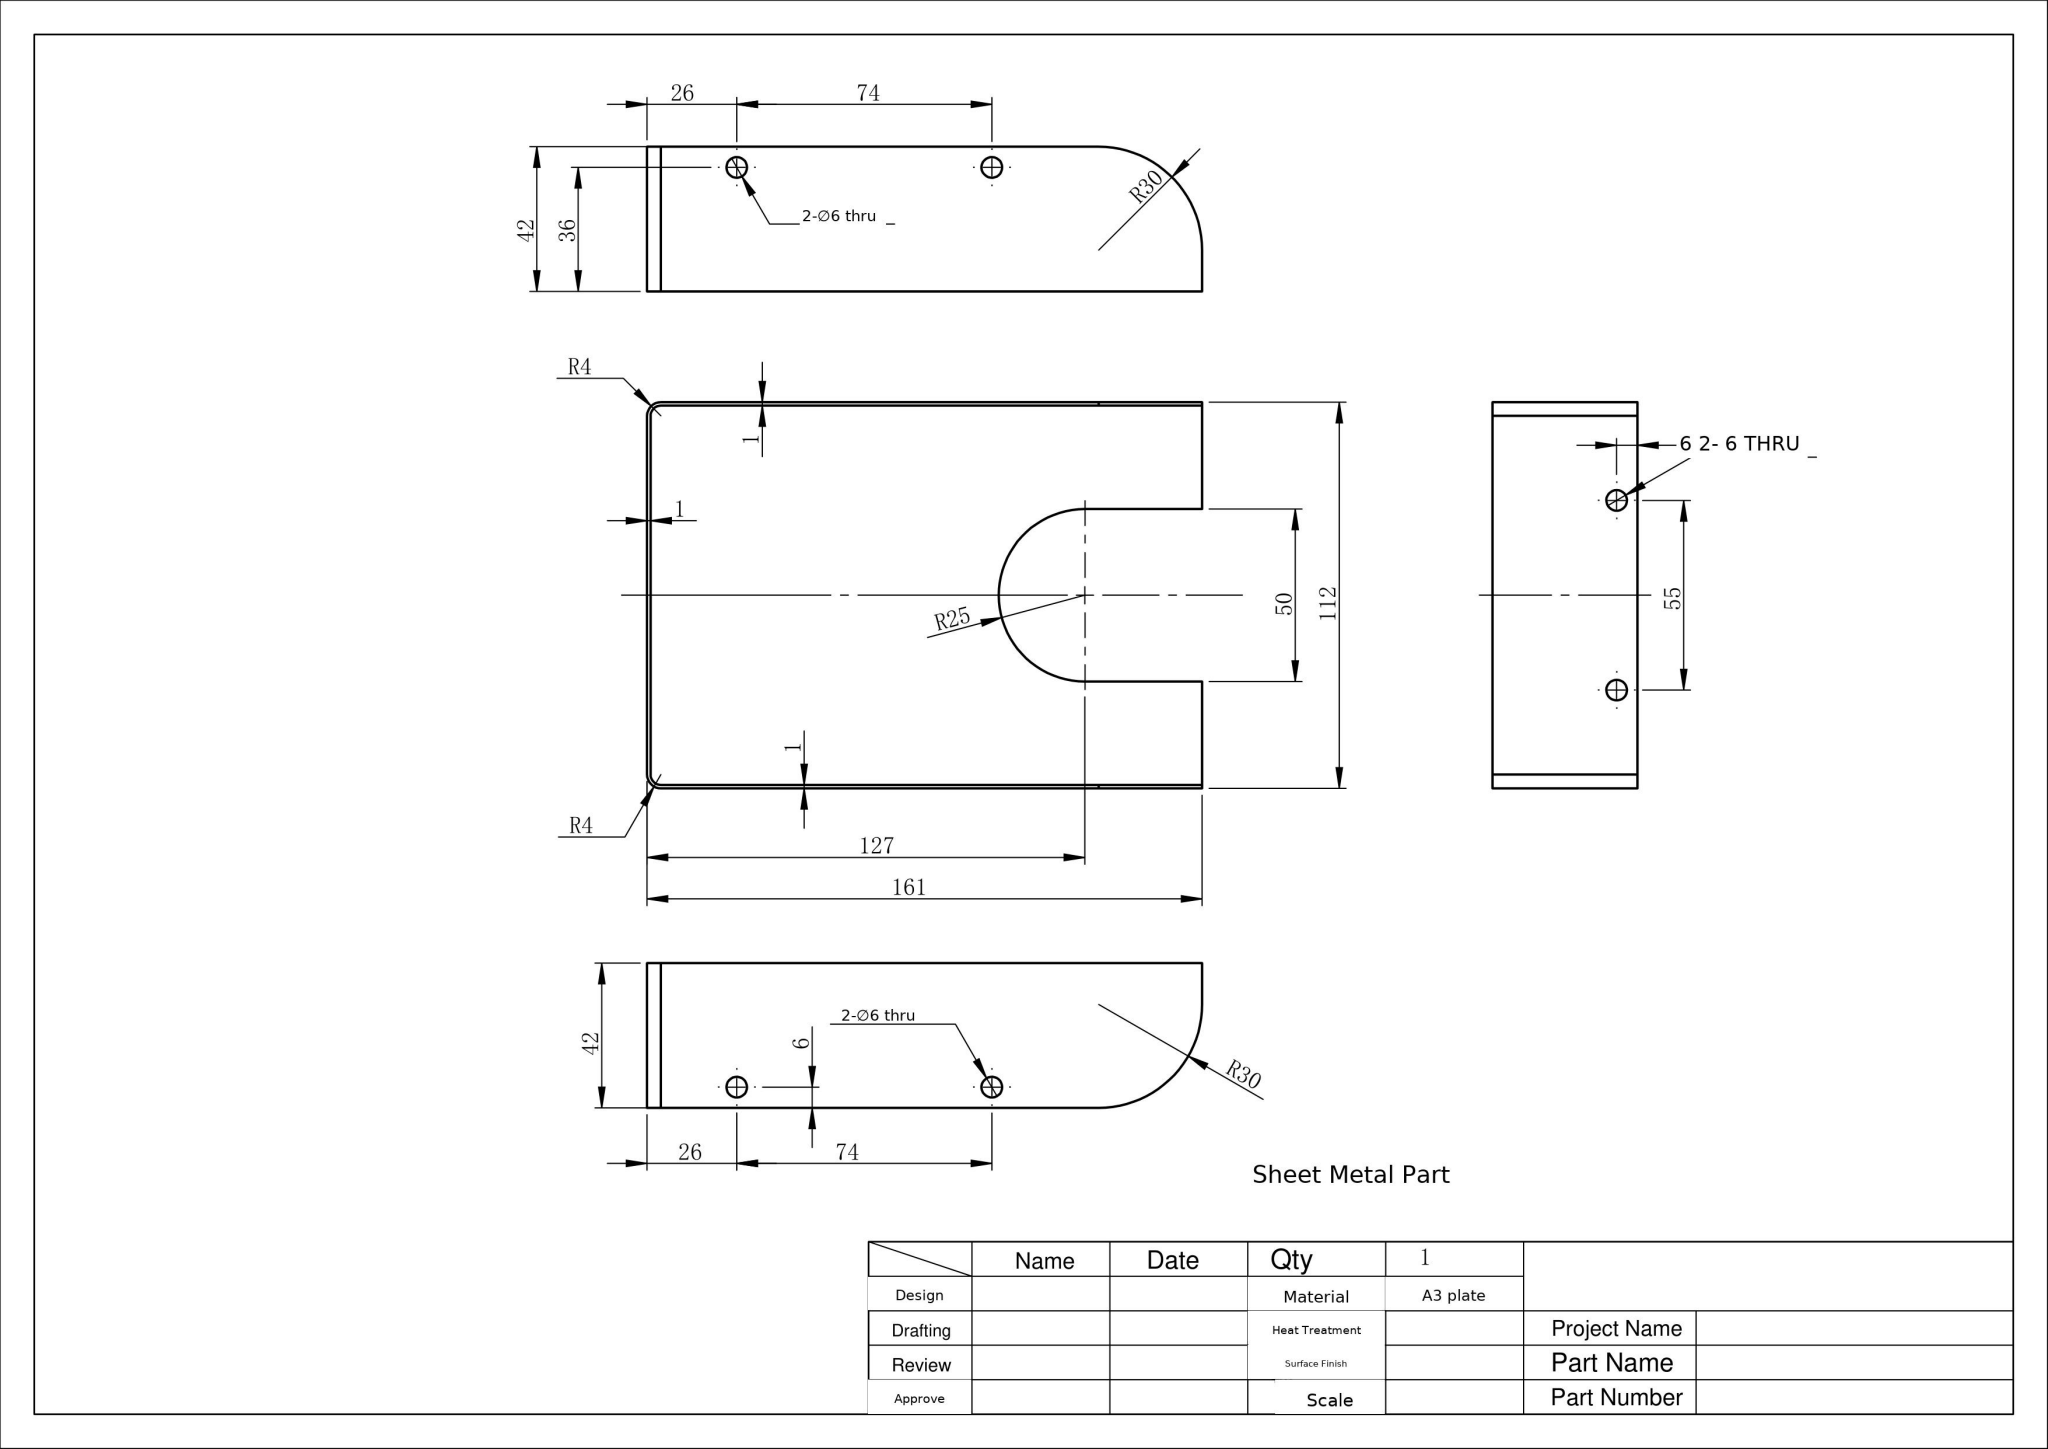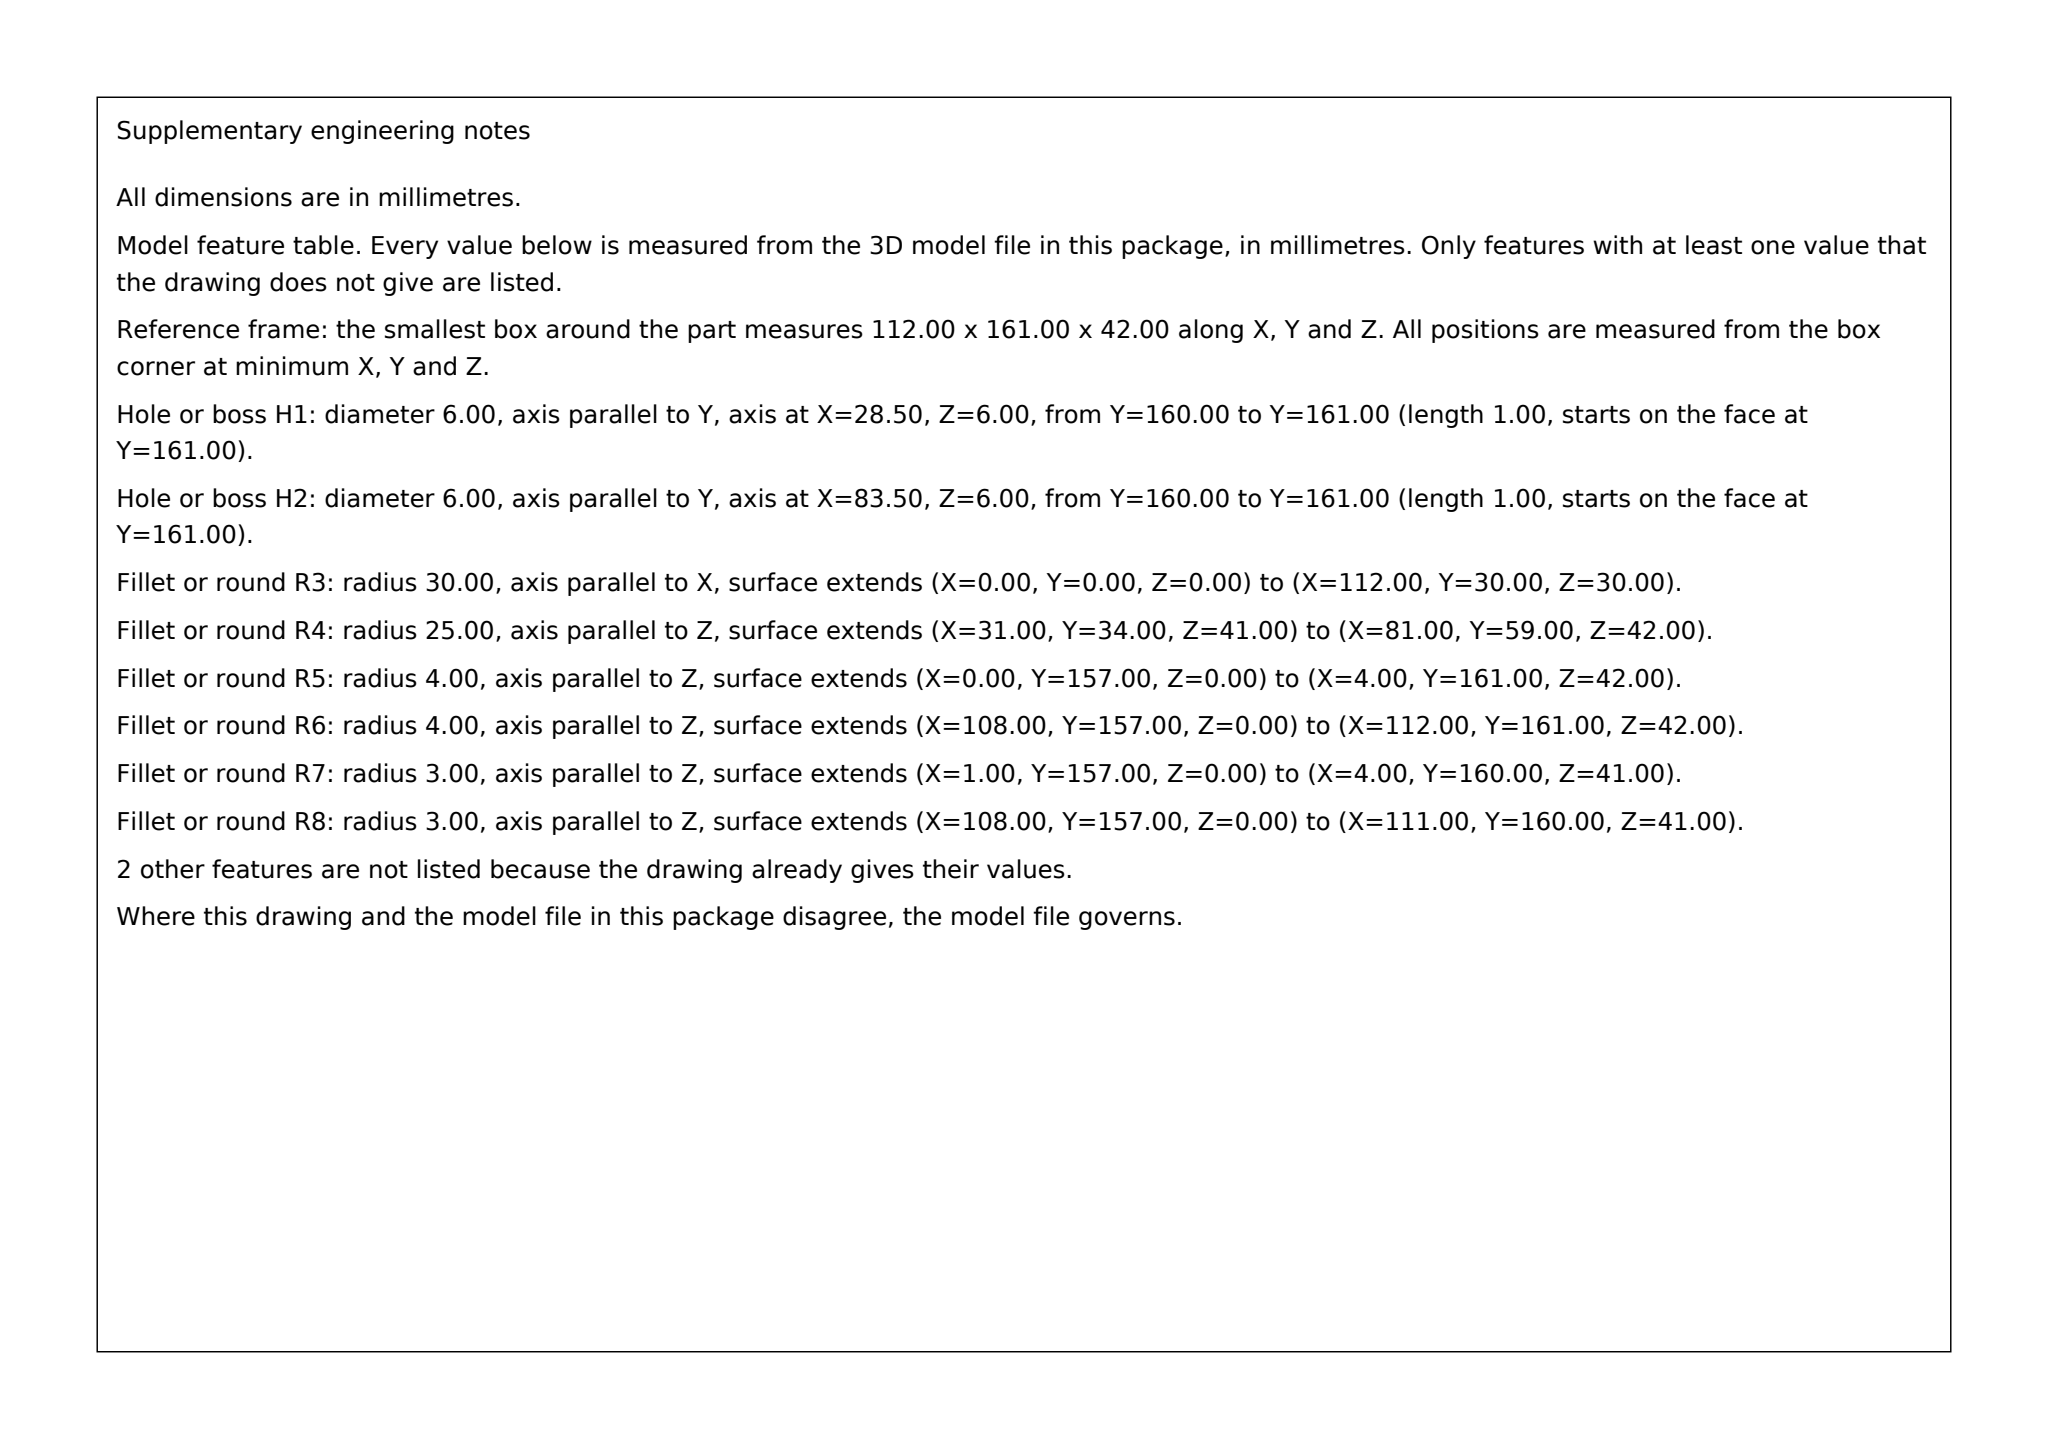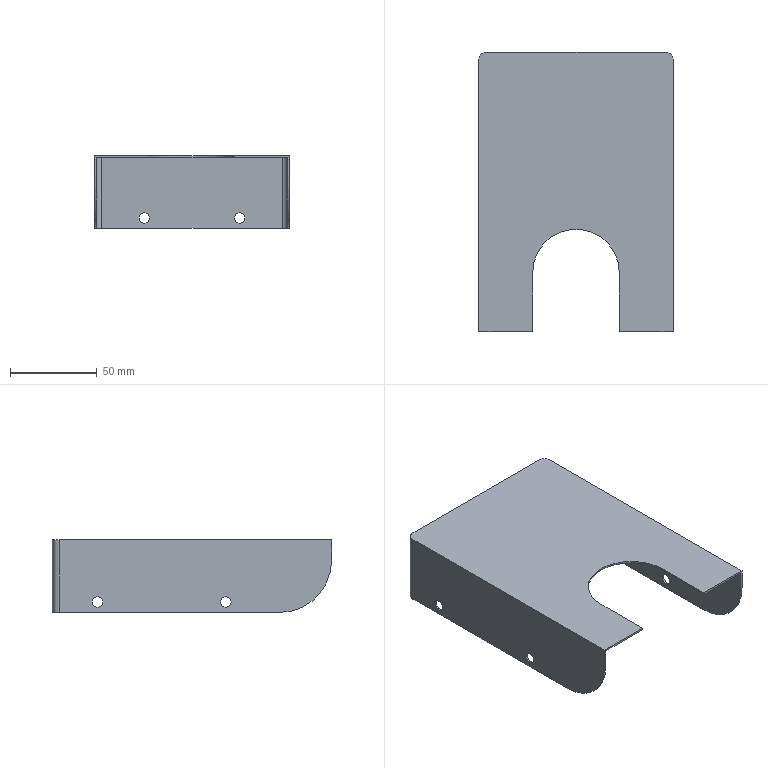Part | SolidWorks | mm | material A3 plate | 1 solid | 32 faces | box 112 x 161 x 42 mm | volume 32376 mm3 | cylinder 19 | plane 13 | commonest cylinder face diameters 6 x14 8 x2 60 x2 50 x1
build123d program:
from build123d import *

# Parameters (mm, degrees)
SKETCH1_W          = 110
SKETCH1_H          = 160
EXTRUDE1_DEPTH     = 1
EXTRUDE2_DEPTH     = 42
FILLET1_R          = 3
FILLET2_R          = 4
SKETCH3_R          = 3
CUT_EXTRUDE1_DEPTH = 32
SKETCH4_R          = 3
CUT_EXTRUDE2_DEPTH = 201.365
CUT_EXTRUDE3_DEPTH = 200.807
FILLET3_R          = 30


with BuildPart() as part:
    # Sketch1 → Extrude1 (new body)
    with BuildSketch(Plane.XY):
        with Locations((55, 80)):
            Rectangle(SKETCH1_W, SKETCH1_H)
    extrude(amount=EXTRUDE1_DEPTH)

    # Sketch2 → Extrude2 (add)
    with BuildSketch(Plane.XY.offset(1)):
        Polygon((0, 0), (-1, 0), (-1, 161), (111, 161), (111, 0), (110, 0), (110, 160), (0, 160), align=None)
    extrude(amount=-EXTRUDE2_DEPTH)

    # Fillet1
    fillet1_edges = [part.edges().sort_by_distance(p)[0] for p in [
        (0, 160, -20.5),
        (110, 160, -20.5),
    ]]
    fillet(fillet1_edges, radius=FILLET1_R)

    # Fillet2
    fillet2_edges = [part.edges().sort_by_distance(p)[0] for p in [
        (-1, 161, -20),
        (111, 161, -20),
    ]]
    fillet(fillet2_edges, radius=FILLET2_R)

    # Sketch3 → Cut-Extrude1 (cut)
    with BuildSketch(Plane(origin=(0, 161, 0), x_dir=(1, 0, 0), z_dir=(0, 1, 0))):
        with Locations(Location((27.5, 35, 0), (0, 0, 180))):
            Circle(SKETCH3_R)
        with Locations(Location((82.5, 35, 0), (0, 0, 180))):
            Circle(SKETCH3_R)
    extrude(amount=-CUT_EXTRUDE1_DEPTH, mode=Mode.SUBTRACT)

    # Sketch4 → Cut-Extrude2 (cut, through all)
    with BuildSketch(Plane.ZY.offset(1)):
        with Locations(Location((-35, 135, 0), (0, 0, 270))):
            Circle(SKETCH4_R)
        with Locations(Location((-35, 61, 0), (0, 0, 270))):
            Circle(SKETCH4_R)
    extrude(amount=-CUT_EXTRUDE2_DEPTH, mode=Mode.SUBTRACT)

    # Sketch5 → Cut-Extrude3 (cut, through all)
    with BuildSketch(Plane(origin=(0, 0, 0), x_dir=(-1, 0, 0), z_dir=(0, 0, -1))):
        with BuildLine():
            Line((-80, -17.994), (-30, -17.994))
            Line((-30, -17.994), (-30, 34))
            ThreePointArc((-30, 34), (-55, 59), (-80, 34))
            Line((-80, 34), (-80, -17.994))
        make_face()
    extrude(amount=-CUT_EXTRUDE3_DEPTH, mode=Mode.SUBTRACT)

    # Fillet3
    fillet3_edges = [part.edges().sort_by_distance(p)[0] for p in [
        (-0.5, 0, -41),
        (110.5, 0, -41),
    ]]
    fillet(fillet3_edges, radius=FILLET3_R)


solid = part.part